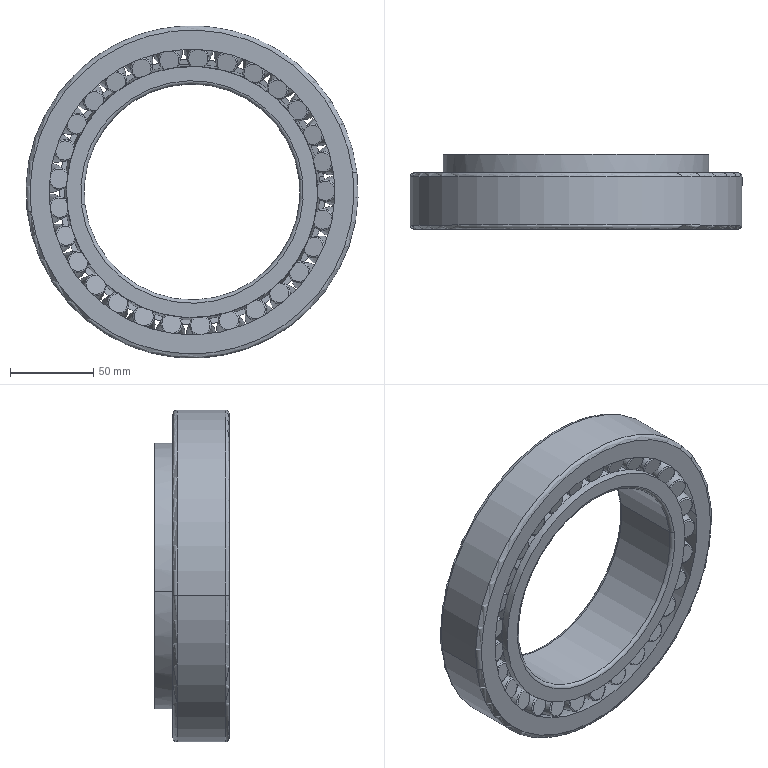Component | SolidWorks | tapered roller bearings gb-10 | 1 solid | 260 faces | box 200 x 45 x 200 mm | volume 562972 mm3 | torus 124 | cone 66 | plane 62 | cylinder 8 | commonest cylinder face diameters 200 x2 151.219 x2 160.004 x2 130 x2